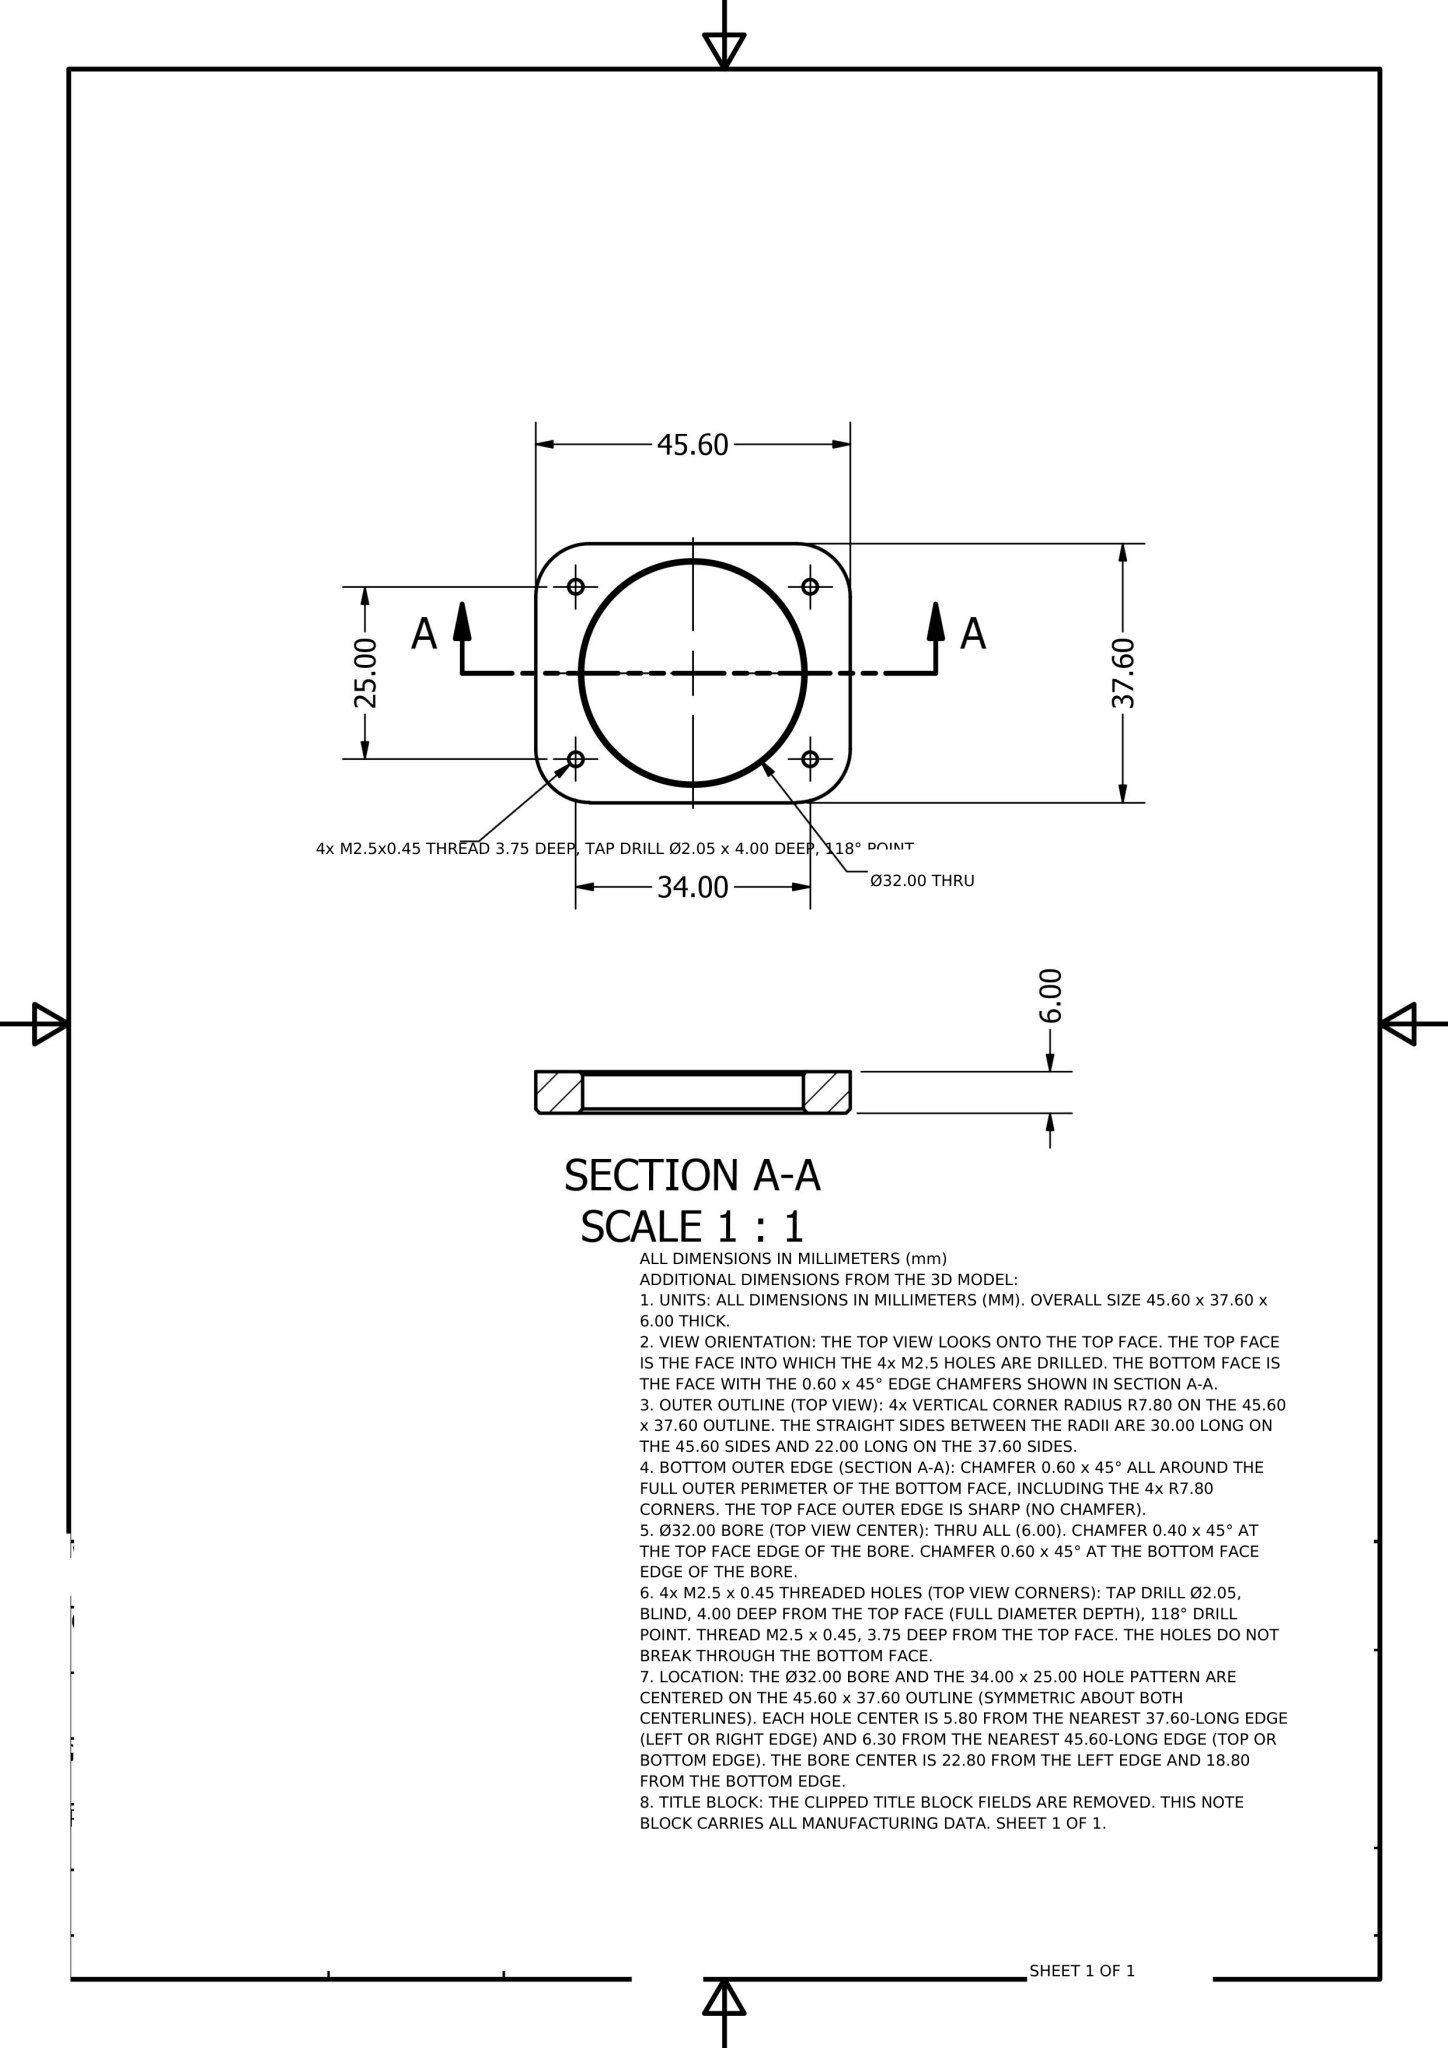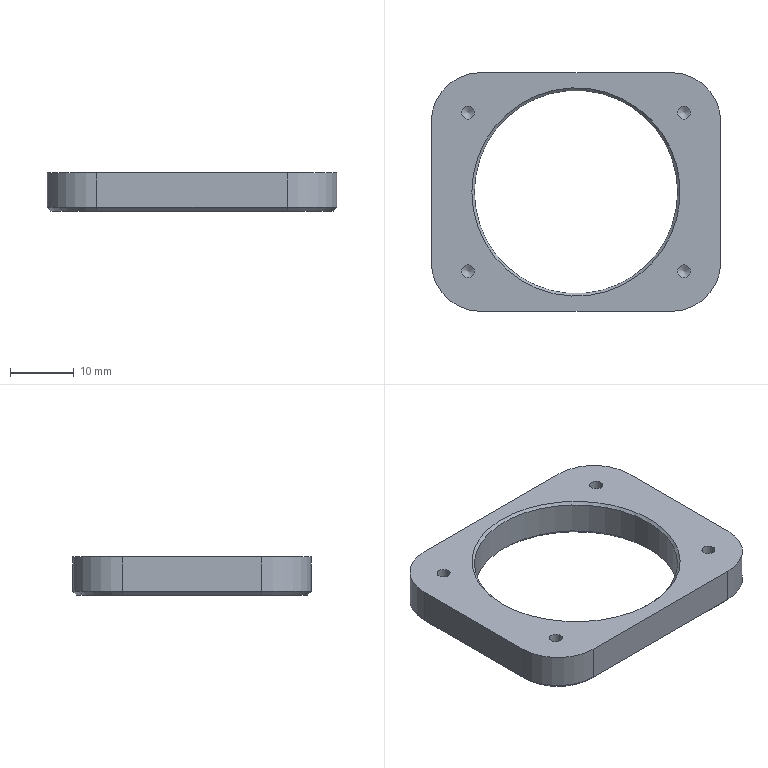Part | NX | mm | 1 solid | 29 faces | box 45.6 x 37.6 x 6 mm | volume 5039 mm3 | plane 10 | cone 10 | cylinder 9 | commonest cylinder face diameters 15.6 x4 2.05 x4 32 x1
STEP:
#1=COLOUR_RGB('',0.8667,0.9098,1.);
#2=FILL_AREA_STYLE_COLOUR('',#1);
#3=FILL_AREA_STYLE('',(#2));
#4=SURFACE_STYLE_FILL_AREA(#3);
#5=SURFACE_STYLE_TRANSPARENT(0.);
#6=SURFACE_STYLE_RENDERING_WITH_PROPERTIES($,#1,(#5));
#7=SURFACE_SIDE_STYLE('',(#4,#6));
#8=SURFACE_STYLE_USAGE(.BOTH.,#7);
#9=PRESENTATION_STYLE_ASSIGNMENT((#8));
#10=CARTESIAN_POINT('',(0.874,0.4528,-2.913));
#11=VERTEX_POINT('',#10);
#12=CARTESIAN_POINT('',(0.874,0.4528,-3.126));
#13=VERTEX_POINT('',#12);
#14=CARTESIAN_POINT('',(0.874,0.4528,-2.913));
#15=DIRECTION('',(0.,0.,-1.));
#16=VECTOR('',#15,0.2126);
#17=LINE('',#14,#16);
#18=EDGE_CURVE('',#11,#13,#17,.T.);
#19=ORIENTED_EDGE('',*,*,#18,.T.);
#20=CARTESIAN_POINT('',(1.181,0.1457,-3.126));
#21=VERTEX_POINT('',#20);
#22=CARTESIAN_POINT('',(1.181,0.4528,-3.126));
#23=DIRECTION('',(0.,0.,-1.));
#24=DIRECTION('',(-1.,0.,0.));
#25=AXIS2_PLACEMENT_3D('',#22,#23,#24);
#26=CIRCLE('',#25,0.3071);
#27=EDGE_CURVE('',#13,#21,#26,.F.);
#28=ORIENTED_EDGE('',*,*,#27,.T.);
#29=CARTESIAN_POINT('',(1.181,0.1457,-2.913));
#30=VERTEX_POINT('',#29);
#31=CARTESIAN_POINT('',(1.181,0.1457,-2.913));
#32=DIRECTION('',(0.,0.,-1.));
#33=VECTOR('',#32,0.2126);
#34=LINE('',#31,#33);
#35=EDGE_CURVE('',#30,#21,#34,.T.);
#36=ORIENTED_EDGE('',*,*,#35,.F.);
#37=CARTESIAN_POINT('',(1.181,0.4528,-2.913));
#38=DIRECTION('',(0.,0.,-1.));
#39=DIRECTION('',(-1.,0.,0.));
#40=AXIS2_PLACEMENT_3D('',#37,#38,#39);
#41=CIRCLE('',#40,0.3071);
#42=EDGE_CURVE('',#30,#11,#41,.T.);
#43=ORIENTED_EDGE('',*,*,#42,.T.);
#44=EDGE_LOOP('',(#19,#28,#36,#43));
#45=FACE_OUTER_BOUND('',#44,.T.);
#46=CARTESIAN_POINT('',(1.181,0.4528,-2.913));
#47=DIRECTION('',(0.,0.,-1.));
#48=DIRECTION('',(-1.,0.,0.));
#49=AXIS2_PLACEMENT_3D('',#46,#47,#48);
#50=CYLINDRICAL_SURFACE('',#49,0.3071);
#51=ADVANCED_FACE('',(#45),#50,.T.);
#52=STYLED_ITEM('',(#9),#51);
#53=ORIENTED_EDGE('',*,*,#35,.T.);
#54=CARTESIAN_POINT('',(2.362,0.1457,-3.126));
#55=VERTEX_POINT('',#54);
#56=CARTESIAN_POINT('',(1.181,0.1457,-3.126));
#57=DIRECTION('',(1.,0.,0.));
#58=VECTOR('',#57,1.181);
#59=LINE('',#56,#58);
#60=EDGE_CURVE('',#21,#55,#59,.T.);
#61=ORIENTED_EDGE('',*,*,#60,.T.);
#62=CARTESIAN_POINT('',(2.362,0.1457,-2.913));
#63=VERTEX_POINT('',#62);
#64=CARTESIAN_POINT('',(2.362,0.1457,-2.913));
#65=DIRECTION('',(0.,0.,-1.));
#66=VECTOR('',#65,0.2126);
#67=LINE('',#64,#66);
#68=EDGE_CURVE('',#63,#55,#67,.T.);
#69=ORIENTED_EDGE('',*,*,#68,.F.);
#70=CARTESIAN_POINT('',(2.362,0.1457,-2.913));
#71=DIRECTION('',(-1.,-0.,0.));
#72=VECTOR('',#71,1.181);
#73=LINE('',#70,#72);
#74=EDGE_CURVE('',#63,#30,#73,.T.);
#75=ORIENTED_EDGE('',*,*,#74,.T.);
#76=EDGE_LOOP('',(#53,#61,#69,#75));
#77=FACE_OUTER_BOUND('',#76,.T.);
#78=CARTESIAN_POINT('',(2.362,0.1457,-2.913));
#79=DIRECTION('',(0.,-1.,0.));
#80=DIRECTION('',(0.,0.,-1.));
#81=AXIS2_PLACEMENT_3D('',#78,#79,#80);
#82=PLANE('',#81);
#83=ADVANCED_FACE('',(#77),#82,.T.);
#84=STYLED_ITEM('',(#9),#83);
#85=ORIENTED_EDGE('',*,*,#68,.T.);
#86=CARTESIAN_POINT('',(2.669,0.4528,-3.126));
#87=VERTEX_POINT('',#86);
#88=CARTESIAN_POINT('',(2.362,0.4528,-3.126));
#89=DIRECTION('',(0.,0.,-1.));
#90=DIRECTION('',(-1.,0.,0.));
#91=AXIS2_PLACEMENT_3D('',#88,#89,#90);
#92=CIRCLE('',#91,0.3071);
#93=EDGE_CURVE('',#55,#87,#92,.F.);
#94=ORIENTED_EDGE('',*,*,#93,.T.);
#95=CARTESIAN_POINT('',(2.669,0.4528,-2.913));
#96=VERTEX_POINT('',#95);
#97=CARTESIAN_POINT('',(2.669,0.4528,-2.913));
#98=DIRECTION('',(0.,0.,-1.));
#99=VECTOR('',#98,0.2126);
#100=LINE('',#97,#99);
#101=EDGE_CURVE('',#96,#87,#100,.T.);
#102=ORIENTED_EDGE('',*,*,#101,.F.);
#103=CARTESIAN_POINT('',(2.362,0.4528,-2.913));
#104=DIRECTION('',(0.,0.,-1.));
#105=DIRECTION('',(-1.,0.,0.));
#106=AXIS2_PLACEMENT_3D('',#103,#104,#105);
#107=CIRCLE('',#106,0.3071);
#108=EDGE_CURVE('',#96,#63,#107,.T.);
#109=ORIENTED_EDGE('',*,*,#108,.T.);
#110=EDGE_LOOP('',(#85,#94,#102,#109));
#111=FACE_OUTER_BOUND('',#110,.T.);
#112=CARTESIAN_POINT('',(2.362,0.4528,-2.913));
#113=DIRECTION('',(0.,0.,-1.));
#114=DIRECTION('',(-1.,0.,0.));
#115=AXIS2_PLACEMENT_3D('',#112,#113,#114);
#116=CYLINDRICAL_SURFACE('',#115,0.3071);
#117=ADVANCED_FACE('',(#111),#116,.T.);
#118=STYLED_ITEM('',(#9),#117);
#119=ORIENTED_EDGE('',*,*,#101,.T.);
#120=CARTESIAN_POINT('',(2.669,1.319,-3.126));
#121=VERTEX_POINT('',#120);
#122=CARTESIAN_POINT('',(2.669,0.4528,-3.126));
#123=DIRECTION('',(0.,1.,0.));
#124=VECTOR('',#123,0.8661);
#125=LINE('',#122,#124);
#126=EDGE_CURVE('',#87,#121,#125,.T.);
#127=ORIENTED_EDGE('',*,*,#126,.T.);
#128=CARTESIAN_POINT('',(2.669,1.319,-2.913));
#129=VERTEX_POINT('',#128);
#130=CARTESIAN_POINT('',(2.669,1.319,-2.913));
#131=DIRECTION('',(0.,0.,-1.));
#132=VECTOR('',#131,0.2126);
#133=LINE('',#130,#132);
#134=EDGE_CURVE('',#129,#121,#133,.T.);
#135=ORIENTED_EDGE('',*,*,#134,.F.);
#136=CARTESIAN_POINT('',(2.669,1.319,-2.913));
#137=DIRECTION('',(0.,-1.,0.));
#138=VECTOR('',#137,0.8661);
#139=LINE('',#136,#138);
#140=EDGE_CURVE('',#129,#96,#139,.T.);
#141=ORIENTED_EDGE('',*,*,#140,.T.);
#142=EDGE_LOOP('',(#119,#127,#135,#141));
#143=FACE_OUTER_BOUND('',#142,.T.);
#144=CARTESIAN_POINT('',(2.669,1.319,-2.913));
#145=DIRECTION('',(1.,0.,0.));
#146=DIRECTION('',(0.,0.,-1.));
#147=AXIS2_PLACEMENT_3D('',#144,#145,#146);
#148=PLANE('',#147);
#149=ADVANCED_FACE('',(#143),#148,.T.);
#150=STYLED_ITEM('',(#9),#149);
#151=ORIENTED_EDGE('',*,*,#134,.T.);
#152=CARTESIAN_POINT('',(2.362,1.626,-3.126));
#153=VERTEX_POINT('',#152);
#154=CARTESIAN_POINT('',(2.362,1.319,-3.126));
#155=DIRECTION('',(0.,0.,-1.));
#156=DIRECTION('',(-1.,0.,0.));
#157=AXIS2_PLACEMENT_3D('',#154,#155,#156);
#158=CIRCLE('',#157,0.3071);
#159=EDGE_CURVE('',#121,#153,#158,.F.);
#160=ORIENTED_EDGE('',*,*,#159,.T.);
#161=CARTESIAN_POINT('',(2.362,1.626,-2.913));
#162=VERTEX_POINT('',#161);
#163=CARTESIAN_POINT('',(2.362,1.626,-2.913));
#164=DIRECTION('',(0.,0.,-1.));
#165=VECTOR('',#164,0.2126);
#166=LINE('',#163,#165);
#167=EDGE_CURVE('',#162,#153,#166,.T.);
#168=ORIENTED_EDGE('',*,*,#167,.F.);
#169=CARTESIAN_POINT('',(2.362,1.319,-2.913));
#170=DIRECTION('',(0.,0.,-1.));
#171=DIRECTION('',(-1.,0.,0.));
#172=AXIS2_PLACEMENT_3D('',#169,#170,#171);
#173=CIRCLE('',#172,0.3071);
#174=EDGE_CURVE('',#162,#129,#173,.T.);
#175=ORIENTED_EDGE('',*,*,#174,.T.);
#176=EDGE_LOOP('',(#151,#160,#168,#175));
#177=FACE_OUTER_BOUND('',#176,.T.);
#178=CARTESIAN_POINT('',(2.362,1.319,-2.913));
#179=DIRECTION('',(0.,0.,-1.));
#180=DIRECTION('',(-1.,0.,0.));
#181=AXIS2_PLACEMENT_3D('',#178,#179,#180);
#182=CYLINDRICAL_SURFACE('',#181,0.3071);
#183=ADVANCED_FACE('',(#177),#182,.T.);
#184=STYLED_ITEM('',(#9),#183);
#185=ORIENTED_EDGE('',*,*,#167,.T.);
#186=CARTESIAN_POINT('',(1.181,1.626,-3.126));
#187=VERTEX_POINT('',#186);
#188=CARTESIAN_POINT('',(2.362,1.626,-3.126));
#189=DIRECTION('',(-1.,0.,0.));
#190=VECTOR('',#189,1.181);
#191=LINE('',#188,#190);
#192=EDGE_CURVE('',#153,#187,#191,.T.);
#193=ORIENTED_EDGE('',*,*,#192,.T.);
#194=CARTESIAN_POINT('',(1.181,1.626,-2.913));
#195=VERTEX_POINT('',#194);
#196=CARTESIAN_POINT('',(1.181,1.626,-2.913));
#197=DIRECTION('',(0.,0.,-1.));
#198=VECTOR('',#197,0.2126);
#199=LINE('',#196,#198);
#200=EDGE_CURVE('',#195,#187,#199,.T.);
#201=ORIENTED_EDGE('',*,*,#200,.F.);
#202=CARTESIAN_POINT('',(1.181,1.626,-2.913));
#203=DIRECTION('',(1.,0.,0.));
#204=VECTOR('',#203,1.181);
#205=LINE('',#202,#204);
#206=EDGE_CURVE('',#195,#162,#205,.T.);
#207=ORIENTED_EDGE('',*,*,#206,.T.);
#208=EDGE_LOOP('',(#185,#193,#201,#207));
#209=FACE_OUTER_BOUND('',#208,.T.);
#210=CARTESIAN_POINT('',(1.181,1.626,-2.913));
#211=DIRECTION('',(0.,1.,0.));
#212=DIRECTION('',(0.,0.,1.));
#213=AXIS2_PLACEMENT_3D('',#210,#211,#212);
#214=PLANE('',#213);
#215=ADVANCED_FACE('',(#209),#214,.T.);
#216=STYLED_ITEM('',(#9),#215);
#217=ORIENTED_EDGE('',*,*,#200,.T.);
#218=CARTESIAN_POINT('',(0.874,1.319,-3.126));
#219=VERTEX_POINT('',#218);
#220=CARTESIAN_POINT('',(1.181,1.319,-3.126));
#221=DIRECTION('',(0.,0.,-1.));
#222=DIRECTION('',(-1.,0.,0.));
#223=AXIS2_PLACEMENT_3D('',#220,#221,#222);
#224=CIRCLE('',#223,0.3071);
#225=EDGE_CURVE('',#187,#219,#224,.F.);
#226=ORIENTED_EDGE('',*,*,#225,.T.);
#227=CARTESIAN_POINT('',(0.874,1.319,-2.913));
#228=VERTEX_POINT('',#227);
#229=CARTESIAN_POINT('',(0.874,1.319,-2.913));
#230=DIRECTION('',(0.,0.,-1.));
#231=VECTOR('',#230,0.2126);
#232=LINE('',#229,#231);
#233=EDGE_CURVE('',#228,#219,#232,.T.);
#234=ORIENTED_EDGE('',*,*,#233,.F.);
#235=CARTESIAN_POINT('',(1.181,1.319,-2.913));
#236=DIRECTION('',(0.,0.,-1.));
#237=DIRECTION('',(-1.,0.,0.));
#238=AXIS2_PLACEMENT_3D('',#235,#236,#237);
#239=CIRCLE('',#238,0.3071);
#240=EDGE_CURVE('',#228,#195,#239,.T.);
#241=ORIENTED_EDGE('',*,*,#240,.T.);
#242=EDGE_LOOP('',(#217,#226,#234,#241));
#243=FACE_OUTER_BOUND('',#242,.T.);
#244=CARTESIAN_POINT('',(1.181,1.319,-2.913));
#245=DIRECTION('',(0.,0.,-1.));
#246=DIRECTION('',(-1.,0.,0.));
#247=AXIS2_PLACEMENT_3D('',#244,#245,#246);
#248=CYLINDRICAL_SURFACE('',#247,0.3071);
#249=ADVANCED_FACE('',(#243),#248,.T.);
#250=STYLED_ITEM('',(#9),#249);
#251=ORIENTED_EDGE('',*,*,#233,.T.);
#252=CARTESIAN_POINT('',(0.874,1.319,-3.126));
#253=DIRECTION('',(0.,-1.,0.));
#254=VECTOR('',#253,0.8661);
#255=LINE('',#252,#254);
#256=EDGE_CURVE('',#219,#13,#255,.T.);
#257=ORIENTED_EDGE('',*,*,#256,.T.);
#258=ORIENTED_EDGE('',*,*,#18,.F.);
#259=CARTESIAN_POINT('',(0.874,0.4528,-2.913));
#260=DIRECTION('',(0.,1.,0.));
#261=VECTOR('',#260,0.8661);
#262=LINE('',#259,#261);
#263=EDGE_CURVE('',#11,#228,#262,.T.);
#264=ORIENTED_EDGE('',*,*,#263,.T.);
#265=EDGE_LOOP('',(#251,#257,#258,#264));
#266=FACE_OUTER_BOUND('',#265,.T.);
#267=CARTESIAN_POINT('',(0.874,0.4528,-2.913));
#268=DIRECTION('',(-1.,0.,0.));
#269=DIRECTION('',(0.,0.,1.));
#270=AXIS2_PLACEMENT_3D('',#267,#268,#269);
#271=PLANE('',#270);
#272=ADVANCED_FACE('',(#266),#271,.T.);
#273=STYLED_ITEM('',(#9),#272);
#274=ORIENTED_EDGE('',*,*,#42,.F.);
#275=ORIENTED_EDGE('',*,*,#74,.F.);
#276=ORIENTED_EDGE('',*,*,#108,.F.);
#277=ORIENTED_EDGE('',*,*,#140,.F.);
#278=ORIENTED_EDGE('',*,*,#174,.F.);
#279=ORIENTED_EDGE('',*,*,#206,.F.);
#280=ORIENTED_EDGE('',*,*,#240,.F.);
#281=ORIENTED_EDGE('',*,*,#263,.F.);
#282=EDGE_LOOP('',(#274,#275,#276,#277,#278,#279,#280,#281));
#283=FACE_OUTER_BOUND('',#282,.T.);
#284=CARTESIAN_POINT('',(1.126,0.8858,-2.913));
#285=VERTEX_POINT('',#284);
#286=CARTESIAN_POINT('',(1.772,0.8858,-2.913));
#287=DIRECTION('',(0.,0.,-1.));
#288=DIRECTION('',(-1.,0.,0.));
#289=AXIS2_PLACEMENT_3D('',#286,#287,#288);
#290=CIRCLE('',#289,0.6457);
#291=EDGE_CURVE('',#285,#285,#290,.T.);
#292=ORIENTED_EDGE('',*,*,#291,.T.);
#293=EDGE_LOOP('',(#292));
#294=FACE_BOUND('',#293,.T.);
#295=CARTESIAN_POINT('',(1.143,1.378,-2.913));
#296=VERTEX_POINT('',#295);
#297=CARTESIAN_POINT('',(1.062,1.378,-2.913));
#298=VERTEX_POINT('',#297);
#299=CARTESIAN_POINT('',(1.102,1.378,-2.913));
#300=DIRECTION('',(0.,0.,1.));
#301=DIRECTION('',(1.,0.,0.));
#302=AXIS2_PLACEMENT_3D('',#299,#300,#301);
#303=CIRCLE('',#302,0.04035);
#304=EDGE_CURVE('',#296,#298,#303,.T.);
#305=ORIENTED_EDGE('',*,*,#304,.F.);
#306=CARTESIAN_POINT('',(1.102,1.378,-2.913));
#307=DIRECTION('',(0.,0.,1.));
#308=DIRECTION('',(1.,0.,0.));
#309=AXIS2_PLACEMENT_3D('',#306,#307,#308);
#310=CIRCLE('',#309,0.04035);
#311=EDGE_CURVE('',#298,#296,#310,.T.);
#312=ORIENTED_EDGE('',*,*,#311,.F.);
#313=EDGE_LOOP('',(#305,#312));
#314=FACE_BOUND('',#313,.T.);
#315=CARTESIAN_POINT('',(2.481,1.378,-2.913));
#316=VERTEX_POINT('',#315);
#317=CARTESIAN_POINT('',(2.401,1.378,-2.913));
#318=VERTEX_POINT('',#317);
#319=CARTESIAN_POINT('',(2.441,1.378,-2.913));
#320=DIRECTION('',(0.,0.,1.));
#321=DIRECTION('',(1.,0.,0.));
#322=AXIS2_PLACEMENT_3D('',#319,#320,#321);
#323=CIRCLE('',#322,0.04035);
#324=EDGE_CURVE('',#316,#318,#323,.T.);
#325=ORIENTED_EDGE('',*,*,#324,.F.);
#326=CARTESIAN_POINT('',(2.441,1.378,-2.913));
#327=DIRECTION('',(0.,0.,1.));
#328=DIRECTION('',(1.,0.,0.));
#329=AXIS2_PLACEMENT_3D('',#326,#327,#328);
#330=CIRCLE('',#329,0.04035);
#331=EDGE_CURVE('',#318,#316,#330,.T.);
#332=ORIENTED_EDGE('',*,*,#331,.F.);
#333=EDGE_LOOP('',(#325,#332));
#334=FACE_BOUND('',#333,.T.);
#335=CARTESIAN_POINT('',(2.481,0.3937,-2.913));
#336=VERTEX_POINT('',#335);
#337=CARTESIAN_POINT('',(2.401,0.3937,-2.913));
#338=VERTEX_POINT('',#337);
#339=CARTESIAN_POINT('',(2.441,0.3937,-2.913));
#340=DIRECTION('',(0.,0.,1.));
#341=DIRECTION('',(1.,0.,0.));
#342=AXIS2_PLACEMENT_3D('',#339,#340,#341);
#343=CIRCLE('',#342,0.04035);
#344=EDGE_CURVE('',#336,#338,#343,.T.);
#345=ORIENTED_EDGE('',*,*,#344,.F.);
#346=CARTESIAN_POINT('',(2.441,0.3937,-2.913));
#347=DIRECTION('',(0.,0.,1.));
#348=DIRECTION('',(1.,0.,0.));
#349=AXIS2_PLACEMENT_3D('',#346,#347,#348);
#350=CIRCLE('',#349,0.04035);
#351=EDGE_CURVE('',#338,#336,#350,.T.);
#352=ORIENTED_EDGE('',*,*,#351,.F.);
#353=EDGE_LOOP('',(#345,#352));
#354=FACE_BOUND('',#353,.T.);
#355=CARTESIAN_POINT('',(1.143,0.3937,-2.913));
#356=VERTEX_POINT('',#355);
#357=CARTESIAN_POINT('',(1.062,0.3937,-2.913));
#358=VERTEX_POINT('',#357);
#359=CARTESIAN_POINT('',(1.102,0.3937,-2.913));
#360=DIRECTION('',(0.,0.,1.));
#361=DIRECTION('',(1.,0.,0.));
#362=AXIS2_PLACEMENT_3D('',#359,#360,#361);
#363=CIRCLE('',#362,0.04035);
#364=EDGE_CURVE('',#356,#358,#363,.T.);
#365=ORIENTED_EDGE('',*,*,#364,.F.);
#366=CARTESIAN_POINT('',(1.102,0.3937,-2.913));
#367=DIRECTION('',(0.,0.,1.));
#368=DIRECTION('',(1.,0.,0.));
#369=AXIS2_PLACEMENT_3D('',#366,#367,#368);
#370=CIRCLE('',#369,0.04035);
#371=EDGE_CURVE('',#358,#356,#370,.T.);
#372=ORIENTED_EDGE('',*,*,#371,.F.);
#373=EDGE_LOOP('',(#365,#372));
#374=FACE_BOUND('',#373,.T.);
#375=CARTESIAN_POINT('',(1.181,0.4528,-2.913));
#376=DIRECTION('',(0.,0.,-1.));
#377=DIRECTION('',(-1.,0.,0.));
#378=AXIS2_PLACEMENT_3D('',#375,#376,#377);
#379=PLANE('',#378);
#380=ADVANCED_FACE('',(#283,#294,#314,#334,#354,#374),#379,.F.);
#381=STYLED_ITEM('',(#9),#380);
#382=CARTESIAN_POINT('',(2.362,0.1693,-3.15));
#383=VERTEX_POINT('',#382);
#384=CARTESIAN_POINT('',(1.181,0.1693,-3.15));
#385=VERTEX_POINT('',#384);
#386=CARTESIAN_POINT('',(2.362,0.1693,-3.15));
#387=DIRECTION('',(-1.,0.,0.));
#388=VECTOR('',#387,1.181);
#389=LINE('',#386,#388);
#390=EDGE_CURVE('',#383,#385,#389,.T.);
#391=ORIENTED_EDGE('',*,*,#390,.T.);
#392=CARTESIAN_POINT('',(0.8976,0.4528,-3.15));
#393=VERTEX_POINT('',#392);
#394=CARTESIAN_POINT('',(1.181,0.4528,-3.15));
#395=DIRECTION('',(0.,0.,-1.));
#396=DIRECTION('',(-1.,0.,0.));
#397=AXIS2_PLACEMENT_3D('',#394,#395,#396);
#398=CIRCLE('',#397,0.2835);
#399=EDGE_CURVE('',#385,#393,#398,.T.);
#400=ORIENTED_EDGE('',*,*,#399,.T.);
#401=CARTESIAN_POINT('',(0.8976,1.319,-3.15));
#402=VERTEX_POINT('',#401);
#403=CARTESIAN_POINT('',(0.8976,0.4528,-3.15));
#404=DIRECTION('',(0.,1.,0.));
#405=VECTOR('',#404,0.8661);
#406=LINE('',#403,#405);
#407=EDGE_CURVE('',#393,#402,#406,.T.);
#408=ORIENTED_EDGE('',*,*,#407,.T.);
#409=CARTESIAN_POINT('',(1.181,1.602,-3.15));
#410=VERTEX_POINT('',#409);
#411=CARTESIAN_POINT('',(1.181,1.319,-3.15));
#412=DIRECTION('',(0.,0.,-1.));
#413=DIRECTION('',(-1.,0.,0.));
#414=AXIS2_PLACEMENT_3D('',#411,#412,#413);
#415=CIRCLE('',#414,0.2835);
#416=EDGE_CURVE('',#402,#410,#415,.T.);
#417=ORIENTED_EDGE('',*,*,#416,.T.);
#418=CARTESIAN_POINT('',(2.362,1.602,-3.15));
#419=VERTEX_POINT('',#418);
#420=CARTESIAN_POINT('',(1.181,1.602,-3.15));
#421=DIRECTION('',(1.,0.,0.));
#422=VECTOR('',#421,1.181);
#423=LINE('',#420,#422);
#424=EDGE_CURVE('',#410,#419,#423,.T.);
#425=ORIENTED_EDGE('',*,*,#424,.T.);
#426=CARTESIAN_POINT('',(2.646,1.319,-3.15));
#427=VERTEX_POINT('',#426);
#428=CARTESIAN_POINT('',(2.362,1.319,-3.15));
#429=DIRECTION('',(0.,0.,-1.));
#430=DIRECTION('',(-1.,0.,0.));
#431=AXIS2_PLACEMENT_3D('',#428,#429,#430);
#432=CIRCLE('',#431,0.2835);
#433=EDGE_CURVE('',#419,#427,#432,.T.);
#434=ORIENTED_EDGE('',*,*,#433,.T.);
#435=CARTESIAN_POINT('',(2.646,0.4528,-3.15));
#436=VERTEX_POINT('',#435);
#437=CARTESIAN_POINT('',(2.646,1.319,-3.15));
#438=DIRECTION('',(0.,-1.,0.));
#439=VECTOR('',#438,0.8661);
#440=LINE('',#437,#439);
#441=EDGE_CURVE('',#427,#436,#440,.T.);
#442=ORIENTED_EDGE('',*,*,#441,.T.);
#443=CARTESIAN_POINT('',(2.362,0.4528,-3.15));
#444=DIRECTION('',(0.,0.,-1.));
#445=DIRECTION('',(-1.,0.,0.));
#446=AXIS2_PLACEMENT_3D('',#443,#444,#445);
#447=CIRCLE('',#446,0.2835);
#448=EDGE_CURVE('',#436,#383,#447,.T.);
#449=ORIENTED_EDGE('',*,*,#448,.T.);
#450=EDGE_LOOP('',(#391,#400,#408,#417,#425,#434,#442,#449));
#451=FACE_OUTER_BOUND('',#450,.T.);
#452=CARTESIAN_POINT('',(1.118,0.8858,-3.15));
#453=VERTEX_POINT('',#452);
#454=CARTESIAN_POINT('',(2.425,0.8858,-3.15));
#455=VERTEX_POINT('',#454);
#456=CARTESIAN_POINT('',(1.772,0.8858,-3.15));
#457=DIRECTION('',(0.,0.,-1.));
#458=DIRECTION('',(-1.,0.,0.));
#459=AXIS2_PLACEMENT_3D('',#456,#457,#458);
#460=CIRCLE('',#459,0.6535);
#461=EDGE_CURVE('',#453,#455,#460,.F.);
#462=ORIENTED_EDGE('',*,*,#461,.T.);
#463=CARTESIAN_POINT('',(1.772,0.8858,-3.15));
#464=DIRECTION('',(0.,0.,-1.));
#465=DIRECTION('',(-1.,0.,0.));
#466=AXIS2_PLACEMENT_3D('',#463,#464,#465);
#467=CIRCLE('',#466,0.6535);
#468=EDGE_CURVE('',#455,#453,#467,.F.);
#469=ORIENTED_EDGE('',*,*,#468,.T.);
#470=EDGE_LOOP('',(#462,#469));
#471=FACE_BOUND('',#470,.T.);
#472=CARTESIAN_POINT('',(1.181,0.4528,-3.15));
#473=DIRECTION('',(0.,0.,-1.));
#474=DIRECTION('',(-1.,0.,0.));
#475=AXIS2_PLACEMENT_3D('',#472,#473,#474);
#476=PLANE('',#475);
#477=ADVANCED_FACE('',(#451,#471),#476,.T.);
#478=STYLED_ITEM('',(#9),#477);
#479=CARTESIAN_POINT('',(1.142,0.8858,-2.929));
#480=VERTEX_POINT('',#479);
#481=CARTESIAN_POINT('',(2.402,0.8858,-2.929));
#482=VERTEX_POINT('',#481);
#483=CARTESIAN_POINT('',(1.772,0.8858,-2.929));
#484=DIRECTION('',(0.,0.,-1.));
#485=DIRECTION('',(-1.,0.,0.));
#486=AXIS2_PLACEMENT_3D('',#483,#484,#485);
#487=CIRCLE('',#486,0.6299);
#488=EDGE_CURVE('',#480,#482,#487,.F.);
#489=ORIENTED_EDGE('',*,*,#488,.T.);
#490=CARTESIAN_POINT('',(2.402,0.8858,-3.126));
#491=VERTEX_POINT('',#490);
#492=CARTESIAN_POINT('',(2.402,0.8858,-2.913));
#493=DIRECTION('',(0.,0.,-1.));
#494=VECTOR('',#493,0.6299);
#495=LINE('',#492,#494);
#496=EDGE_CURVE('',#482,#491,#495,.T.);
#497=ORIENTED_EDGE('',*,*,#496,.T.);
#498=CARTESIAN_POINT('',(1.142,0.8858,-3.126));
#499=VERTEX_POINT('',#498);
#500=CARTESIAN_POINT('',(1.772,0.8858,-3.126));
#501=DIRECTION('',(0.,0.,-1.));
#502=DIRECTION('',(-1.,0.,0.));
#503=AXIS2_PLACEMENT_3D('',#500,#501,#502);
#504=CIRCLE('',#503,0.6299);
#505=EDGE_CURVE('',#491,#499,#504,.T.);
#506=ORIENTED_EDGE('',*,*,#505,.T.);
#507=CARTESIAN_POINT('',(1.772,0.8858,-3.126));
#508=DIRECTION('',(0.,0.,-1.));
#509=DIRECTION('',(-1.,0.,0.));
#510=AXIS2_PLACEMENT_3D('',#507,#508,#509);
#511=CIRCLE('',#510,0.6299);
#512=EDGE_CURVE('',#499,#491,#511,.T.);
#513=ORIENTED_EDGE('',*,*,#512,.T.);
#514=ORIENTED_EDGE('',*,*,#496,.F.);
#515=CARTESIAN_POINT('',(1.772,0.8858,-2.929));
#516=DIRECTION('',(0.,0.,-1.));
#517=DIRECTION('',(-1.,0.,0.));
#518=AXIS2_PLACEMENT_3D('',#515,#516,#517);
#519=CIRCLE('',#518,0.6299);
#520=EDGE_CURVE('',#482,#480,#519,.F.);
#521=ORIENTED_EDGE('',*,*,#520,.T.);
#522=EDGE_LOOP('',(#489,#497,#506,#513,#514,#521));
#523=FACE_OUTER_BOUND('',#522,.T.);
#524=CARTESIAN_POINT('',(1.772,0.8858,-2.913));
#525=DIRECTION('',(0.,0.,-1.));
#526=DIRECTION('',(-1.,0.,0.));
#527=AXIS2_PLACEMENT_3D('',#524,#525,#526);
#528=CYLINDRICAL_SURFACE('',#527,0.6299);
#529=ADVANCED_FACE('',(#523),#528,.F.);
#530=STYLED_ITEM('',(#9),#529);
#531=CARTESIAN_POINT('',(1.102,0.3937,-3.095));
#532=VERTEX_POINT('',#531);
#533=CARTESIAN_POINT('',(1.062,0.3937,-3.071));
#534=VERTEX_POINT('',#533);
#535=CARTESIAN_POINT('',(1.062,0.3937,-3.071));
#536=DIRECTION('',(-0.8572,-0.,0.515));
#537=VECTOR('',#536,0.04035);
#538=LINE('',#535,#537);
#539=EDGE_CURVE('',#532,#534,#538,.T.);
#540=ORIENTED_EDGE('',*,*,#539,.T.);
#541=CARTESIAN_POINT('',(1.143,0.3937,-3.071));
#542=VERTEX_POINT('',#541);
#543=CARTESIAN_POINT('',(1.102,0.3937,-3.071));
#544=DIRECTION('',(0.,0.,1.));
#545=DIRECTION('',(1.,0.,0.));
#546=AXIS2_PLACEMENT_3D('',#543,#544,#545);
#547=CIRCLE('',#546,0.04035);
#548=EDGE_CURVE('',#534,#542,#547,.T.);
#549=ORIENTED_EDGE('',*,*,#548,.T.);
#550=CARTESIAN_POINT('',(1.102,0.3937,-3.071));
#551=DIRECTION('',(0.,0.,1.));
#552=DIRECTION('',(1.,0.,0.));
#553=AXIS2_PLACEMENT_3D('',#550,#551,#552);
#554=CIRCLE('',#553,0.04035);
#555=EDGE_CURVE('',#542,#534,#554,.T.);
#556=ORIENTED_EDGE('',*,*,#555,.T.);
#557=ORIENTED_EDGE('',*,*,#539,.F.);
#558=EDGE_LOOP('',(#540,#549,#556,#557));
#559=FACE_OUTER_BOUND('',#558,.T.);
#560=CARTESIAN_POINT('',(1.102,0.3937,-3.071));
#561=DIRECTION('',(0.,0.,1.));
#562=DIRECTION('',(1.,0.,0.));
#563=AXIS2_PLACEMENT_3D('',#560,#561,#562);
#564=CONICAL_SURFACE('',#563,0.04035,1.03);
#565=ADVANCED_FACE('',(#559),#564,.F.);
#566=STYLED_ITEM('',(#9),#565);
#567=COLOUR_RGB('',0.898,0.9176,0.9294);
#568=FILL_AREA_STYLE_COLOUR('',#567);
#569=FILL_AREA_STYLE('',(#568));
#570=SURFACE_STYLE_FILL_AREA(#569);
#571=SURFACE_STYLE_TRANSPARENT(0.);
#572=SURFACE_STYLE_RENDERING_WITH_PROPERTIES($,#567,(#571));
#573=SURFACE_SIDE_STYLE('',(#570,#572));
#574=SURFACE_STYLE_USAGE(.BOTH.,#573);
#575=PRESENTATION_STYLE_ASSIGNMENT((#574));
#576=ORIENTED_EDGE('',*,*,#555,.F.);
#577=ORIENTED_EDGE('',*,*,#548,.F.);
#578=CARTESIAN_POINT('',(1.062,0.3937,-2.913));
#579=DIRECTION('',(0.,0.,1.));
#580=VECTOR('',#579,0.04035);
#581=LINE('',#578,#580);
#582=EDGE_CURVE('',#534,#358,#581,.T.);
#583=ORIENTED_EDGE('',*,*,#582,.T.);
#584=ORIENTED_EDGE('',*,*,#371,.T.);
#585=ORIENTED_EDGE('',*,*,#364,.T.);
#586=ORIENTED_EDGE('',*,*,#582,.F.);
#587=EDGE_LOOP('',(#576,#577,#583,#584,#585,#586));
#588=FACE_OUTER_BOUND('',#587,.T.);
#589=CARTESIAN_POINT('',(1.102,0.3937,-2.913));
#590=DIRECTION('',(0.,0.,1.));
#591=DIRECTION('',(1.,0.,0.));
#592=AXIS2_PLACEMENT_3D('',#589,#590,#591);
#593=CYLINDRICAL_SURFACE('',#592,0.04035);
#594=ADVANCED_FACE('',(#588),#593,.F.);
#595=STYLED_ITEM('',(#575),#594);
#596=CARTESIAN_POINT('',(2.441,0.3937,-3.095));
#597=VERTEX_POINT('',#596);
#598=CARTESIAN_POINT('',(2.401,0.3937,-3.071));
#599=VERTEX_POINT('',#598);
#600=CARTESIAN_POINT('',(2.401,0.3937,-3.071));
#601=DIRECTION('',(-0.8572,-0.,0.515));
#602=VECTOR('',#601,0.04035);
#603=LINE('',#600,#602);
#604=EDGE_CURVE('',#597,#599,#603,.T.);
#605=ORIENTED_EDGE('',*,*,#604,.T.);
#606=CARTESIAN_POINT('',(2.481,0.3937,-3.071));
#607=VERTEX_POINT('',#606);
#608=CARTESIAN_POINT('',(2.441,0.3937,-3.071));
#609=DIRECTION('',(0.,0.,1.));
#610=DIRECTION('',(1.,0.,0.));
#611=AXIS2_PLACEMENT_3D('',#608,#609,#610);
#612=CIRCLE('',#611,0.04035);
#613=EDGE_CURVE('',#599,#607,#612,.T.);
#614=ORIENTED_EDGE('',*,*,#613,.T.);
#615=CARTESIAN_POINT('',(2.441,0.3937,-3.071));
#616=DIRECTION('',(0.,0.,1.));
#617=DIRECTION('',(1.,0.,0.));
#618=AXIS2_PLACEMENT_3D('',#615,#616,#617);
#619=CIRCLE('',#618,0.04035);
#620=EDGE_CURVE('',#607,#599,#619,.T.);
#621=ORIENTED_EDGE('',*,*,#620,.T.);
#622=ORIENTED_EDGE('',*,*,#604,.F.);
#623=EDGE_LOOP('',(#605,#614,#621,#622));
#624=FACE_OUTER_BOUND('',#623,.T.);
#625=CARTESIAN_POINT('',(2.441,0.3937,-3.071));
#626=DIRECTION('',(0.,0.,1.));
#627=DIRECTION('',(1.,0.,0.));
#628=AXIS2_PLACEMENT_3D('',#625,#626,#627);
#629=CONICAL_SURFACE('',#628,0.04035,1.03);
#630=ADVANCED_FACE('',(#624),#629,.F.);
#631=STYLED_ITEM('',(#9),#630);
#632=ORIENTED_EDGE('',*,*,#620,.F.);
#633=ORIENTED_EDGE('',*,*,#613,.F.);
#634=CARTESIAN_POINT('',(2.401,0.3937,-2.913));
#635=DIRECTION('',(0.,0.,1.));
#636=VECTOR('',#635,0.04035);
#637=LINE('',#634,#636);
#638=EDGE_CURVE('',#599,#338,#637,.T.);
#639=ORIENTED_EDGE('',*,*,#638,.T.);
#640=ORIENTED_EDGE('',*,*,#351,.T.);
#641=ORIENTED_EDGE('',*,*,#344,.T.);
#642=ORIENTED_EDGE('',*,*,#638,.F.);
#643=EDGE_LOOP('',(#632,#633,#639,#640,#641,#642));
#644=FACE_OUTER_BOUND('',#643,.T.);
#645=CARTESIAN_POINT('',(2.441,0.3937,-2.913));
#646=DIRECTION('',(0.,0.,1.));
#647=DIRECTION('',(1.,0.,0.));
#648=AXIS2_PLACEMENT_3D('',#645,#646,#647);
#649=CYLINDRICAL_SURFACE('',#648,0.04035);
#650=ADVANCED_FACE('',(#644),#649,.F.);
#651=STYLED_ITEM('',(#575),#650);
#652=CARTESIAN_POINT('',(2.441,1.378,-3.095));
#653=VERTEX_POINT('',#652);
#654=CARTESIAN_POINT('',(2.401,1.378,-3.071));
#655=VERTEX_POINT('',#654);
#656=CARTESIAN_POINT('',(2.401,1.378,-3.071));
#657=DIRECTION('',(-0.8572,-0.,0.515));
#658=VECTOR('',#657,0.04035);
#659=LINE('',#656,#658);
#660=EDGE_CURVE('',#653,#655,#659,.T.);
#661=ORIENTED_EDGE('',*,*,#660,.T.);
#662=CARTESIAN_POINT('',(2.481,1.378,-3.071));
#663=VERTEX_POINT('',#662);
#664=CARTESIAN_POINT('',(2.441,1.378,-3.071));
#665=DIRECTION('',(0.,0.,1.));
#666=DIRECTION('',(1.,0.,0.));
#667=AXIS2_PLACEMENT_3D('',#664,#665,#666);
#668=CIRCLE('',#667,0.04035);
#669=EDGE_CURVE('',#655,#663,#668,.T.);
#670=ORIENTED_EDGE('',*,*,#669,.T.);
#671=CARTESIAN_POINT('',(2.441,1.378,-3.071));
#672=DIRECTION('',(0.,0.,1.));
#673=DIRECTION('',(1.,0.,0.));
#674=AXIS2_PLACEMENT_3D('',#671,#672,#673);
#675=CIRCLE('',#674,0.04035);
#676=EDGE_CURVE('',#663,#655,#675,.T.);
#677=ORIENTED_EDGE('',*,*,#676,.T.);
#678=ORIENTED_EDGE('',*,*,#660,.F.);
#679=EDGE_LOOP('',(#661,#670,#677,#678));
#680=FACE_OUTER_BOUND('',#679,.T.);
#681=CARTESIAN_POINT('',(2.441,1.378,-3.071));
#682=DIRECTION('',(0.,0.,1.));
#683=DIRECTION('',(1.,0.,0.));
#684=AXIS2_PLACEMENT_3D('',#681,#682,#683);
#685=CONICAL_SURFACE('',#684,0.04035,1.03);
#686=ADVANCED_FACE('',(#680),#685,.F.);
#687=STYLED_ITEM('',(#9),#686);
#688=ORIENTED_EDGE('',*,*,#676,.F.);
#689=ORIENTED_EDGE('',*,*,#669,.F.);
#690=CARTESIAN_POINT('',(2.401,1.378,-2.913));
#691=DIRECTION('',(0.,0.,1.));
#692=VECTOR('',#691,0.04035);
#693=LINE('',#690,#692);
#694=EDGE_CURVE('',#655,#318,#693,.T.);
#695=ORIENTED_EDGE('',*,*,#694,.T.);
#696=ORIENTED_EDGE('',*,*,#331,.T.);
#697=ORIENTED_EDGE('',*,*,#324,.T.);
#698=ORIENTED_EDGE('',*,*,#694,.F.);
#699=EDGE_LOOP('',(#688,#689,#695,#696,#697,#698));
#700=FACE_OUTER_BOUND('',#699,.T.);
#701=CARTESIAN_POINT('',(2.441,1.378,-2.913));
#702=DIRECTION('',(0.,0.,1.));
#703=DIRECTION('',(1.,0.,0.));
#704=AXIS2_PLACEMENT_3D('',#701,#702,#703);
#705=CYLINDRICAL_SURFACE('',#704,0.04035);
#706=ADVANCED_FACE('',(#700),#705,.F.);
#707=STYLED_ITEM('',(#575),#706);
#708=CARTESIAN_POINT('',(1.102,1.378,-3.095));
#709=VERTEX_POINT('',#708);
#710=CARTESIAN_POINT('',(1.062,1.378,-3.071));
#711=VERTEX_POINT('',#710);
#712=CARTESIAN_POINT('',(1.062,1.378,-3.071));
#713=DIRECTION('',(-0.8572,-0.,0.515));
#714=VECTOR('',#713,0.04035);
#715=LINE('',#712,#714);
#716=EDGE_CURVE('',#709,#711,#715,.T.);
#717=ORIENTED_EDGE('',*,*,#716,.T.);
#718=CARTESIAN_POINT('',(1.143,1.378,-3.071));
#719=VERTEX_POINT('',#718);
#720=CARTESIAN_POINT('',(1.102,1.378,-3.071));
#721=DIRECTION('',(0.,0.,1.));
#722=DIRECTION('',(1.,0.,0.));
#723=AXIS2_PLACEMENT_3D('',#720,#721,#722);
#724=CIRCLE('',#723,0.04035);
#725=EDGE_CURVE('',#711,#719,#724,.T.);
#726=ORIENTED_EDGE('',*,*,#725,.T.);
#727=CARTESIAN_POINT('',(1.102,1.378,-3.071));
#728=DIRECTION('',(0.,0.,1.));
#729=DIRECTION('',(1.,0.,0.));
#730=AXIS2_PLACEMENT_3D('',#727,#728,#729);
#731=CIRCLE('',#730,0.04035);
#732=EDGE_CURVE('',#719,#711,#731,.T.);
#733=ORIENTED_EDGE('',*,*,#732,.T.);
#734=ORIENTED_EDGE('',*,*,#716,.F.);
#735=EDGE_LOOP('',(#717,#726,#733,#734));
#736=FACE_OUTER_BOUND('',#735,.T.);
#737=CARTESIAN_POINT('',(1.102,1.378,-3.071));
#738=DIRECTION('',(0.,0.,1.));
#739=DIRECTION('',(1.,0.,0.));
#740=AXIS2_PLACEMENT_3D('',#737,#738,#739);
#741=CONICAL_SURFACE('',#740,0.04035,1.03);
#742=ADVANCED_FACE('',(#736),#741,.F.);
#743=STYLED_ITEM('',(#9),#742);
#744=ORIENTED_EDGE('',*,*,#732,.F.);
#745=ORIENTED_EDGE('',*,*,#725,.F.);
#746=CARTESIAN_POINT('',(1.062,1.378,-2.913));
#747=DIRECTION('',(0.,0.,1.));
#748=VECTOR('',#747,0.04035);
#749=LINE('',#746,#748);
#750=EDGE_CURVE('',#711,#298,#749,.T.);
#751=ORIENTED_EDGE('',*,*,#750,.T.);
#752=ORIENTED_EDGE('',*,*,#311,.T.);
#753=ORIENTED_EDGE('',*,*,#304,.T.);
#754=ORIENTED_EDGE('',*,*,#750,.F.);
#755=EDGE_LOOP('',(#744,#745,#751,#752,#753,#754));
#756=FACE_OUTER_BOUND('',#755,.T.);
#757=CARTESIAN_POINT('',(1.102,1.378,-2.913));
#758=DIRECTION('',(0.,0.,1.));
#759=DIRECTION('',(1.,0.,0.));
#760=AXIS2_PLACEMENT_3D('',#757,#758,#759);
#761=CYLINDRICAL_SURFACE('',#760,0.04035);
#762=ADVANCED_FACE('',(#756),#761,.F.);
#763=STYLED_ITEM('',(#575),#762);
#764=CARTESIAN_POINT('',(2.362,1.626,-3.126));
#765=DIRECTION('',(0.,-0.7071,-0.7071));
#766=VECTOR('',#765,0.03341);
#767=LINE('',#764,#766);
#768=EDGE_CURVE('',#153,#419,#767,.T.);
#769=ORIENTED_EDGE('',*,*,#768,.F.);
#770=ORIENTED_EDGE('',*,*,#159,.F.);
#771=CARTESIAN_POINT('',(2.646,1.319,-3.15));
#772=DIRECTION('',(0.7071,0.,0.7071));
#773=VECTOR('',#772,0.03341);
#774=LINE('',#771,#773);
#775=EDGE_CURVE('',#427,#121,#774,.T.);
#776=ORIENTED_EDGE('',*,*,#775,.F.);
#777=ORIENTED_EDGE('',*,*,#433,.F.);
#778=EDGE_LOOP('',(#769,#770,#776,#777));
#779=FACE_OUTER_BOUND('',#778,.T.);
#780=CARTESIAN_POINT('',(2.362,1.319,-3.15));
#781=DIRECTION('',(0.,0.,1.));
#782=DIRECTION('',(1.,0.,0.));
#783=AXIS2_PLACEMENT_3D('',#780,#781,#782);
#784=CONICAL_SURFACE('',#783,0.2835,0.7854);
#785=ADVANCED_FACE('',(#779),#784,.T.);
#786=STYLED_ITEM('',(#9),#785);
#787=ORIENTED_EDGE('',*,*,#775,.T.);
#788=ORIENTED_EDGE('',*,*,#126,.F.);
#789=CARTESIAN_POINT('',(2.646,0.4528,-3.15));
#790=DIRECTION('',(0.7071,0.,0.7071));
#791=VECTOR('',#790,0.03341);
#792=LINE('',#789,#791);
#793=EDGE_CURVE('',#436,#87,#792,.T.);
#794=ORIENTED_EDGE('',*,*,#793,.F.);
#795=ORIENTED_EDGE('',*,*,#441,.F.);
#796=EDGE_LOOP('',(#787,#788,#794,#795));
#797=FACE_OUTER_BOUND('',#796,.T.);
#798=CARTESIAN_POINT('',(2.646,0.4528,-3.15));
#799=DIRECTION('',(-0.7071,0.,0.7071));
#800=DIRECTION('',(0.7071,0.,0.7071));
#801=AXIS2_PLACEMENT_3D('',#798,#799,#800);
#802=PLANE('',#801);
#803=ADVANCED_FACE('',(#797),#802,.F.);
#804=STYLED_ITEM('',(#9),#803);
#805=ORIENTED_EDGE('',*,*,#768,.T.);
#806=ORIENTED_EDGE('',*,*,#424,.F.);
#807=CARTESIAN_POINT('',(1.181,1.626,-3.126));
#808=DIRECTION('',(0.,-0.7071,-0.7071));
#809=VECTOR('',#808,0.03341);
#810=LINE('',#807,#809);
#811=EDGE_CURVE('',#187,#410,#810,.T.);
#812=ORIENTED_EDGE('',*,*,#811,.F.);
#813=ORIENTED_EDGE('',*,*,#192,.F.);
#814=EDGE_LOOP('',(#805,#806,#812,#813));
#815=FACE_OUTER_BOUND('',#814,.T.);
#816=CARTESIAN_POINT('',(1.181,1.602,-3.15));
#817=DIRECTION('',(-0.,-0.7071,0.7071));
#818=DIRECTION('',(1.,0.,0.));
#819=AXIS2_PLACEMENT_3D('',#816,#817,#818);
#820=PLANE('',#819);
#821=ADVANCED_FACE('',(#815),#820,.F.);
#822=STYLED_ITEM('',(#9),#821);
#823=ORIENTED_EDGE('',*,*,#793,.T.);
#824=ORIENTED_EDGE('',*,*,#93,.F.);
#825=CARTESIAN_POINT('',(2.362,0.1693,-3.15));
#826=DIRECTION('',(0.,-0.7071,0.7071));
#827=VECTOR('',#826,0.03341);
#828=LINE('',#825,#827);
#829=EDGE_CURVE('',#383,#55,#828,.T.);
#830=ORIENTED_EDGE('',*,*,#829,.F.);
#831=ORIENTED_EDGE('',*,*,#448,.F.);
#832=EDGE_LOOP('',(#823,#824,#830,#831));
#833=FACE_OUTER_BOUND('',#832,.T.);
#834=CARTESIAN_POINT('',(2.362,0.4528,-3.15));
#835=DIRECTION('',(0.,0.,1.));
#836=DIRECTION('',(1.,0.,0.));
#837=AXIS2_PLACEMENT_3D('',#834,#835,#836);
#838=CONICAL_SURFACE('',#837,0.2835,0.7854);
#839=ADVANCED_FACE('',(#833),#838,.T.);
#840=STYLED_ITEM('',(#9),#839);
#841=ORIENTED_EDGE('',*,*,#811,.T.);
#842=ORIENTED_EDGE('',*,*,#416,.F.);
#843=CARTESIAN_POINT('',(0.874,1.319,-3.126));
#844=DIRECTION('',(0.7071,0.,-0.7071));
#845=VECTOR('',#844,0.03341);
#846=LINE('',#843,#845);
#847=EDGE_CURVE('',#219,#402,#846,.T.);
#848=ORIENTED_EDGE('',*,*,#847,.F.);
#849=ORIENTED_EDGE('',*,*,#225,.F.);
#850=EDGE_LOOP('',(#841,#842,#848,#849));
#851=FACE_OUTER_BOUND('',#850,.T.);
#852=CARTESIAN_POINT('',(1.181,1.319,-3.15));
#853=DIRECTION('',(0.,0.,1.));
#854=DIRECTION('',(1.,0.,0.));
#855=AXIS2_PLACEMENT_3D('',#852,#853,#854);
#856=CONICAL_SURFACE('',#855,0.2835,0.7854);
#857=ADVANCED_FACE('',(#851),#856,.T.);
#858=STYLED_ITEM('',(#9),#857);
#859=ORIENTED_EDGE('',*,*,#829,.T.);
#860=ORIENTED_EDGE('',*,*,#60,.F.);
#861=CARTESIAN_POINT('',(1.181,0.1693,-3.15));
#862=DIRECTION('',(0.,-0.7071,0.7071));
#863=VECTOR('',#862,0.03341);
#864=LINE('',#861,#863);
#865=EDGE_CURVE('',#385,#21,#864,.T.);
#866=ORIENTED_EDGE('',*,*,#865,.F.);
#867=ORIENTED_EDGE('',*,*,#390,.F.);
#868=EDGE_LOOP('',(#859,#860,#866,#867));
#869=FACE_OUTER_BOUND('',#868,.T.);
#870=CARTESIAN_POINT('',(1.181,0.1693,-3.15));
#871=DIRECTION('',(-0.,0.7071,0.7071));
#872=DIRECTION('',(1.,0.,0.));
#873=AXIS2_PLACEMENT_3D('',#870,#871,#872);
#874=PLANE('',#873);
#875=ADVANCED_FACE('',(#869),#874,.F.);
#876=STYLED_ITEM('',(#9),#875);
#877=ORIENTED_EDGE('',*,*,#847,.T.);
#878=ORIENTED_EDGE('',*,*,#407,.F.);
#879=CARTESIAN_POINT('',(0.874,0.4528,-3.126));
#880=DIRECTION('',(0.7071,0.,-0.7071));
#881=VECTOR('',#880,0.03341);
#882=LINE('',#879,#881);
#883=EDGE_CURVE('',#13,#393,#882,.T.);
#884=ORIENTED_EDGE('',*,*,#883,.F.);
#885=ORIENTED_EDGE('',*,*,#256,.F.);
#886=EDGE_LOOP('',(#877,#878,#884,#885));
#887=FACE_OUTER_BOUND('',#886,.T.);
#888=CARTESIAN_POINT('',(0.8976,0.4528,-3.15));
#889=DIRECTION('',(0.7071,0.,0.7071));
#890=DIRECTION('',(0.7071,0.,-0.7071));
#891=AXIS2_PLACEMENT_3D('',#888,#889,#890);
#892=PLANE('',#891);
#893=ADVANCED_FACE('',(#887),#892,.F.);
#894=STYLED_ITEM('',(#9),#893);
#895=ORIENTED_EDGE('',*,*,#865,.T.);
#896=ORIENTED_EDGE('',*,*,#27,.F.);
#897=ORIENTED_EDGE('',*,*,#883,.T.);
#898=ORIENTED_EDGE('',*,*,#399,.F.);
#899=EDGE_LOOP('',(#895,#896,#897,#898));
#900=FACE_OUTER_BOUND('',#899,.T.);
#901=CARTESIAN_POINT('',(1.181,0.4528,-3.15));
#902=DIRECTION('',(0.,0.,1.));
#903=DIRECTION('',(1.,0.,0.));
#904=AXIS2_PLACEMENT_3D('',#901,#902,#903);
#905=CONICAL_SURFACE('',#904,0.2835,0.7854);
#906=ADVANCED_FACE('',(#900),#905,.T.);
#907=STYLED_ITEM('',(#9),#906);
#908=ORIENTED_EDGE('',*,*,#512,.F.);
#909=ORIENTED_EDGE('',*,*,#505,.F.);
#910=CARTESIAN_POINT('',(2.402,0.8858,-3.126));
#911=DIRECTION('',(0.7071,-0.,-0.7071));
#912=VECTOR('',#911,0.6299);
#913=LINE('',#910,#912);
#914=EDGE_CURVE('',#491,#455,#913,.T.);
#915=ORIENTED_EDGE('',*,*,#914,.T.);
#916=ORIENTED_EDGE('',*,*,#461,.F.);
#917=ORIENTED_EDGE('',*,*,#468,.F.);
#918=ORIENTED_EDGE('',*,*,#914,.F.);
#919=EDGE_LOOP('',(#908,#909,#915,#916,#917,#918));
#920=FACE_OUTER_BOUND('',#919,.T.);
#921=CARTESIAN_POINT('',(1.772,0.8858,-3.126));
#922=DIRECTION('',(0.,0.,-1.));
#923=DIRECTION('',(-1.,0.,0.));
#924=AXIS2_PLACEMENT_3D('',#921,#922,#923);
#925=CONICAL_SURFACE('',#924,0.6299,0.7854);
#926=ADVANCED_FACE('',(#920),#925,.F.);
#927=STYLED_ITEM('',(#9),#926);
#928=ORIENTED_EDGE('',*,*,#488,.F.);
#929=CARTESIAN_POINT('',(1.126,0.8858,-2.913));
#930=DIRECTION('',(-0.7071,-0.,0.7071));
#931=VECTOR('',#930,0.6457);
#932=LINE('',#929,#931);
#933=EDGE_CURVE('',#480,#285,#932,.T.);
#934=ORIENTED_EDGE('',*,*,#933,.T.);
#935=ORIENTED_EDGE('',*,*,#291,.F.);
#936=ORIENTED_EDGE('',*,*,#933,.F.);
#937=ORIENTED_EDGE('',*,*,#520,.F.);
#938=EDGE_LOOP('',(#928,#934,#935,#936,#937));
#939=FACE_OUTER_BOUND('',#938,.T.);
#940=CARTESIAN_POINT('',(1.772,0.8858,-2.913));
#941=DIRECTION('',(0.,0.,1.));
#942=DIRECTION('',(1.,0.,0.));
#943=AXIS2_PLACEMENT_3D('',#940,#941,#942);
#944=CONICAL_SURFACE('',#943,0.6457,0.7854);
#945=ADVANCED_FACE('',(#939),#944,.F.);
#946=STYLED_ITEM('',(#9),#945);
#947=COLOUR_RGB('',0.749,0.749,0.749);
#948=FILL_AREA_STYLE_COLOUR('',#947);
#949=FILL_AREA_STYLE('',(#948));
#950=SURFACE_STYLE_FILL_AREA(#949);
#951=SURFACE_STYLE_TRANSPARENT(0.);
#952=SURFACE_STYLE_RENDERING_WITH_PROPERTIES($,#947,(#951));
#953=SURFACE_SIDE_STYLE('',(#950,#952));
#954=SURFACE_STYLE_USAGE(.BOTH.,#953);
#955=PRESENTATION_STYLE_ASSIGNMENT((#954));
#956=CLOSED_SHELL('',(#51,#83,#117,#149,#183,#215,#249,#272,#380,#477,#529,#565,#594,#630,#650,#686,#706,#742,#762,#785,#803,#821,#839,#857,#875,#893,#906,#926,#945));
#957=MANIFOLD_SOLID_BREP('',#956);
#958=STYLED_ITEM('',(#955),#957);
#959=(LENGTH_UNIT()NAMED_UNIT(*)SI_UNIT(.MILLI.,.METRE.));
#960=LENGTH_MEASURE_WITH_UNIT(LENGTH_MEASURE(25.4),#959);
#961=DIMENSIONAL_EXPONENTS(1.,0.,0.,0.,0.,0.,0.);
#962=(CONVERSION_BASED_UNIT('',#960)LENGTH_UNIT()NAMED_UNIT(#961));
#963=UNCERTAINTY_MEASURE_WITH_UNIT(LENGTH_MEASURE(0.0003937),#962,'','');
#964=(NAMED_UNIT(*)PLANE_ANGLE_UNIT()SI_UNIT($,.RADIAN.));
#965=(NAMED_UNIT(*)SI_UNIT($,.STERADIAN.)SOLID_ANGLE_UNIT());
#966=(GEOMETRIC_REPRESENTATION_CONTEXT(3)GLOBAL_UNCERTAINTY_ASSIGNED_CONTEXT((#963))GLOBAL_UNIT_ASSIGNED_CONTEXT((#962,#964,#965))REPRESENTATION_CONTEXT('',''));
#967=MECHANICAL_DESIGN_GEOMETRIC_PRESENTATION_REPRESENTATION('',(#52,#84,#118,#150,#184,#216,#250,#273,#381,#478,#530,#566,#595,#631,#651,#687,#707,#743,#763,#786,#804,#822,#840,#858,#876,#894,#907,#927,#946,#958),#966);
#968=CARTESIAN_POINT('',(0.,0.,0.));
#969=DIRECTION('',(0.,0.,1.));
#970=DIRECTION('',(1.,0.,0.));
#971=AXIS2_PLACEMENT_3D('',#968,#969,#970);
#972=UNCERTAINTY_MEASURE_WITH_UNIT(LENGTH_MEASURE(0.0003937),#962,'','');
#973=(GEOMETRIC_REPRESENTATION_CONTEXT(3)GLOBAL_UNCERTAINTY_ASSIGNED_CONTEXT((#972))GLOBAL_UNIT_ASSIGNED_CONTEXT((#962,#964,#965))REPRESENTATION_CONTEXT('',''));
#974=SHAPE_REPRESENTATION('',(#971),#973);
#975=ADVANCED_BREP_SHAPE_REPRESENTATION('',(#957),#973);
#976=SHAPE_REPRESENTATION_RELATIONSHIP('','',#974,#975);
#977=DESCRIPTIVE_REPRESENTATION_ITEM('','');
#978=REPRESENTATION('',(#977),#973);
#979=(MASS_UNIT()NAMED_UNIT(*)SI_UNIT($,.GRAM.));
#980=DERIVED_UNIT_ELEMENT(#979,1.);
#981=(LENGTH_UNIT()NAMED_UNIT(*)SI_UNIT(.CENTI.,.METRE.));
#982=DERIVED_UNIT_ELEMENT(#981,3.);
#983=DERIVED_UNIT((#980,#982));
#984=MEASURE_REPRESENTATION_ITEM('',POSITIVE_RATIO_MEASURE(1.),#983);
#985=REPRESENTATION('',(#984),#973);